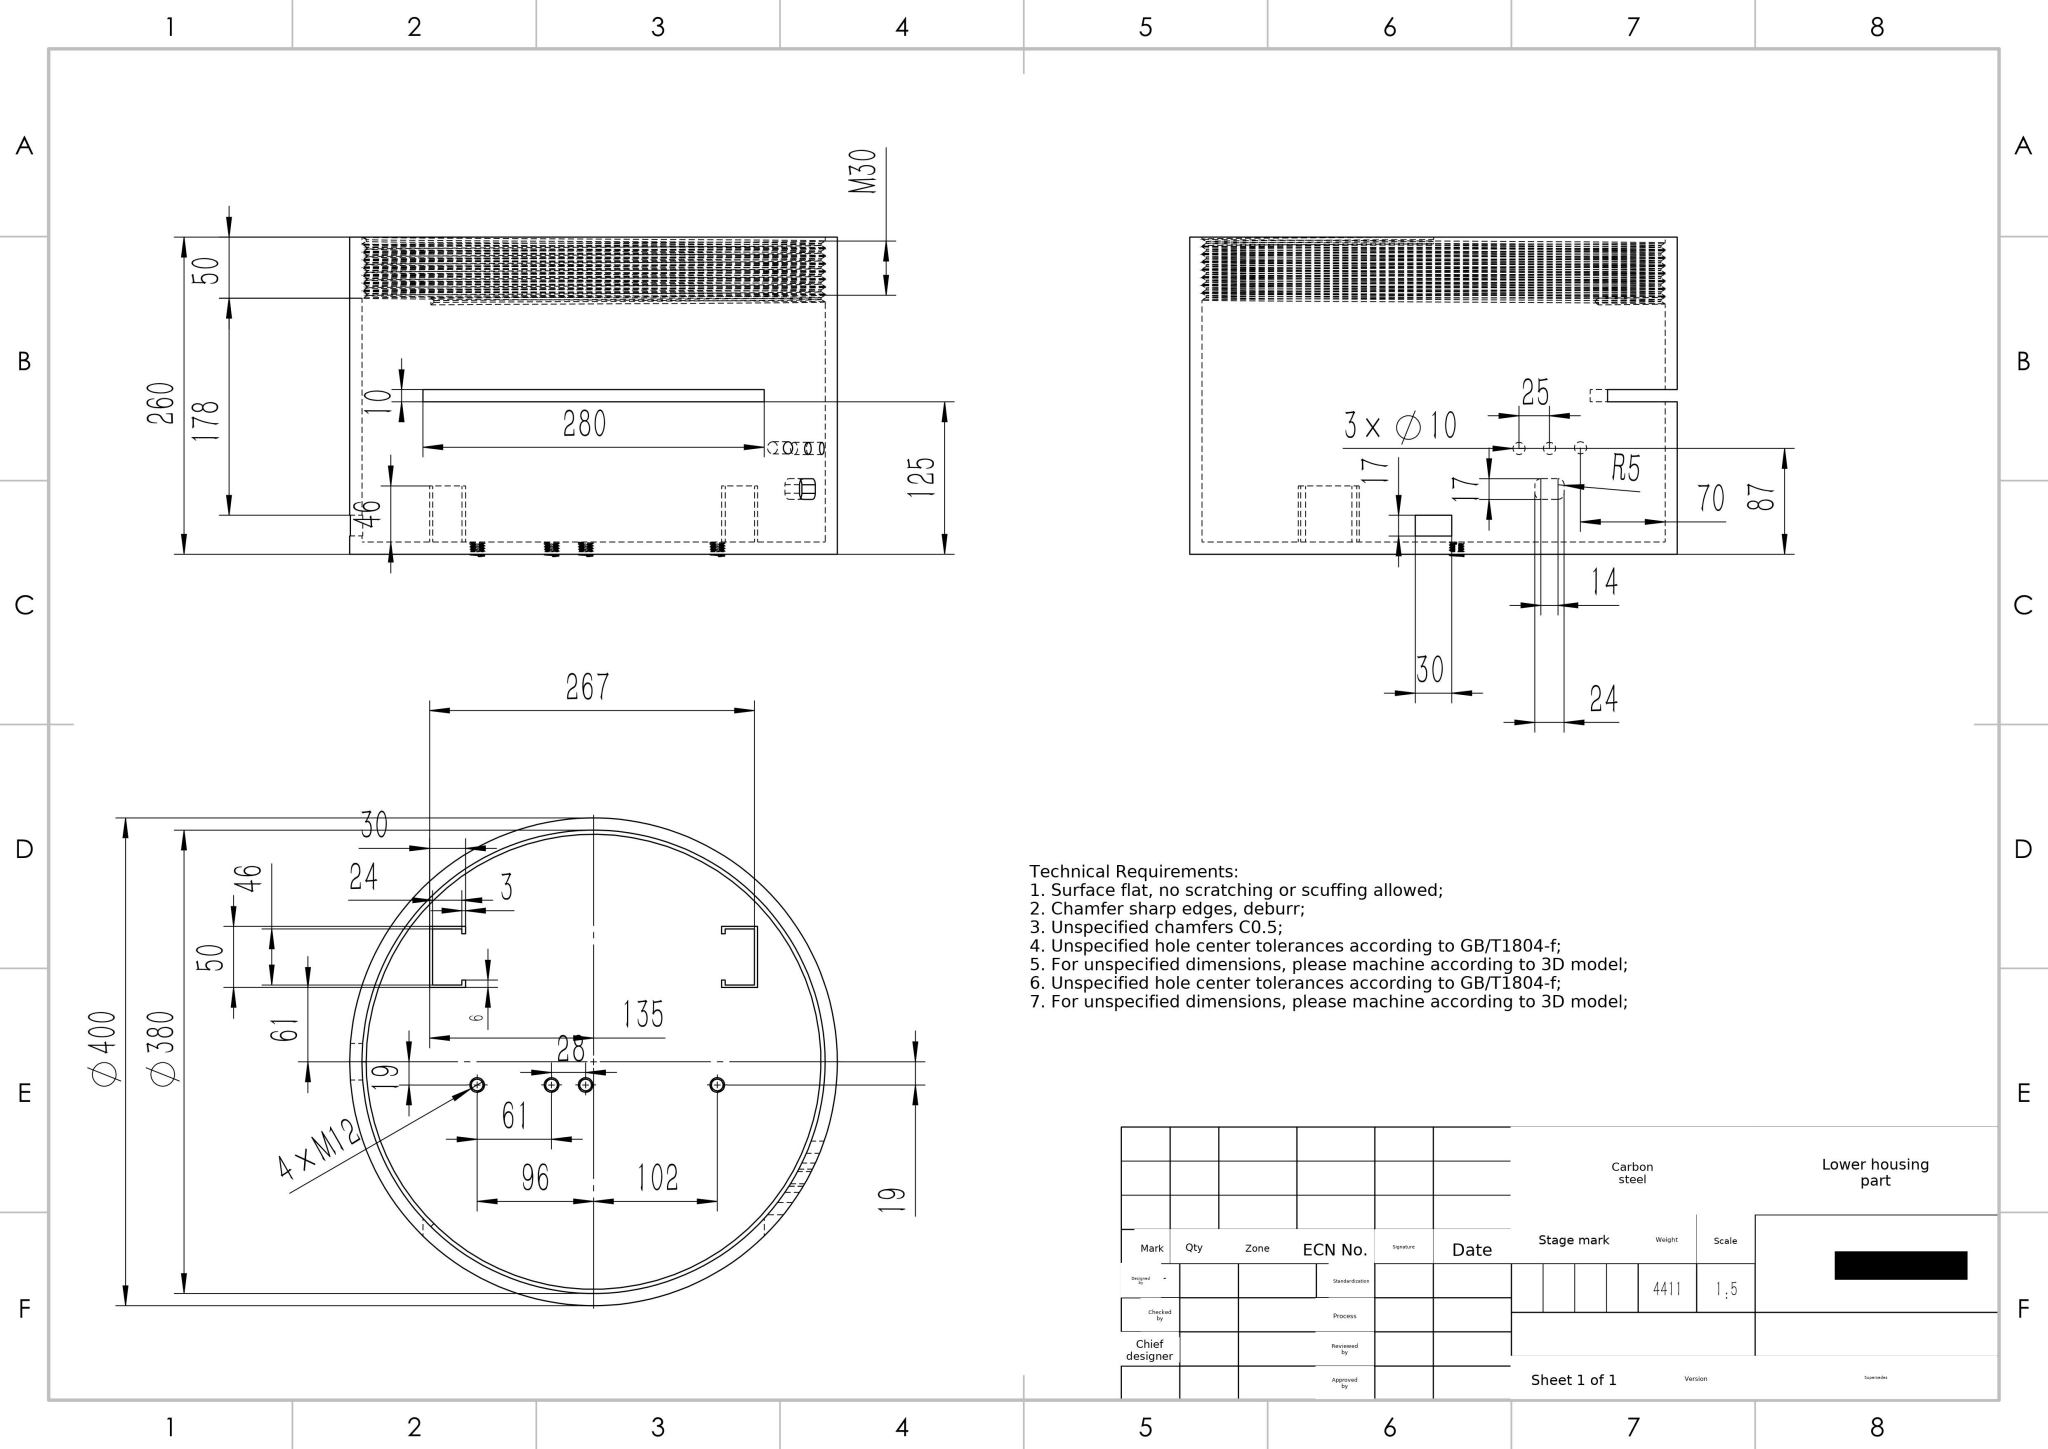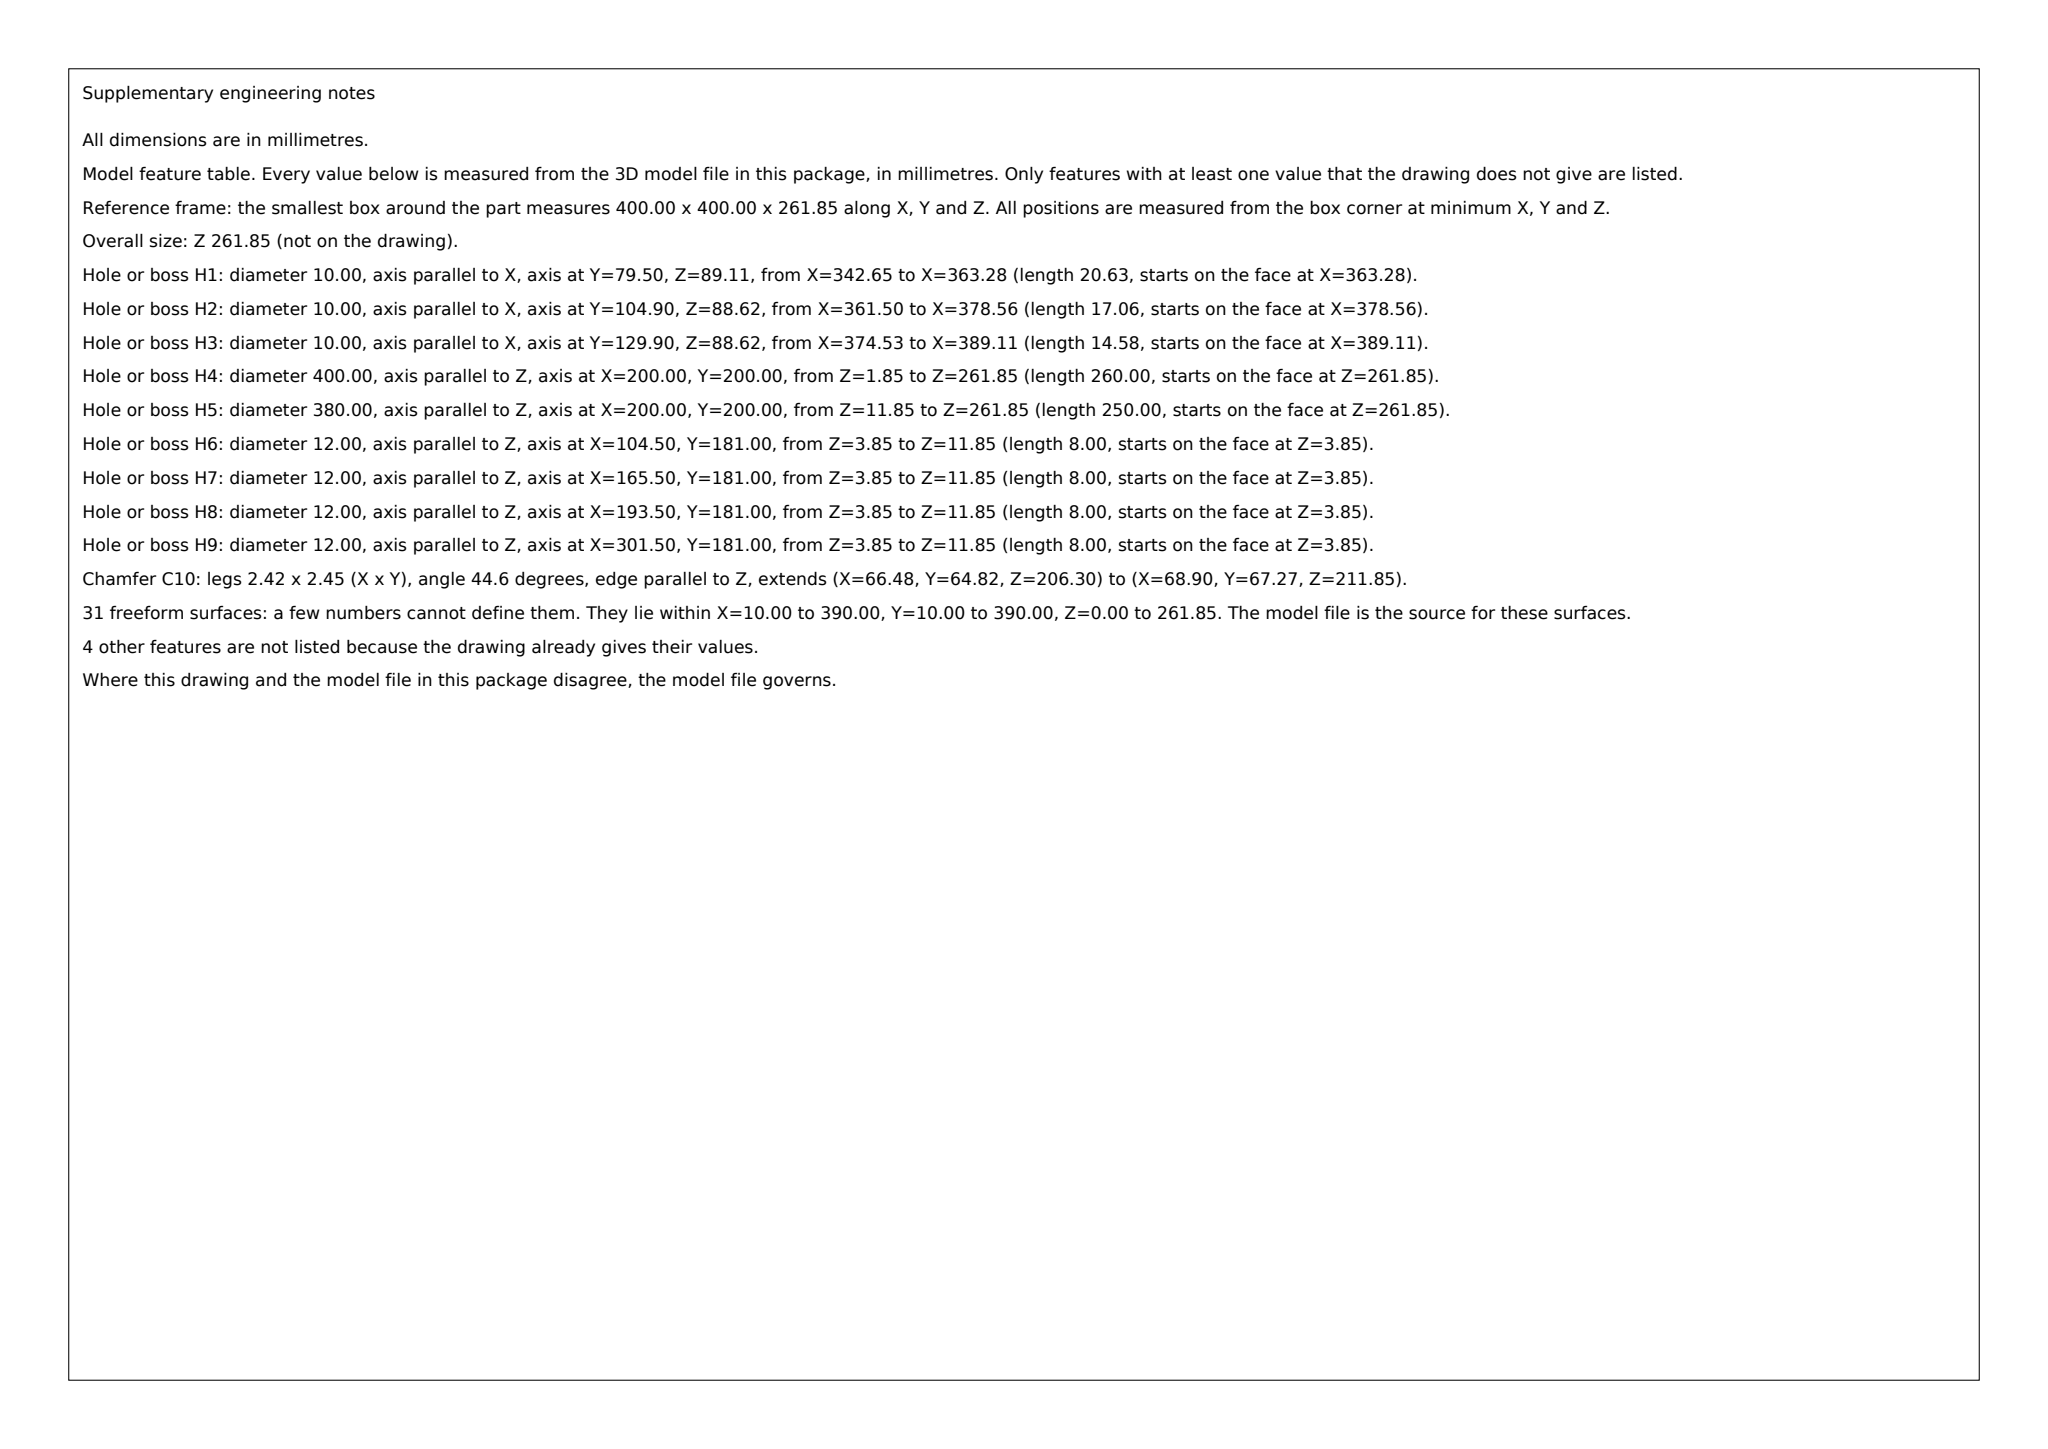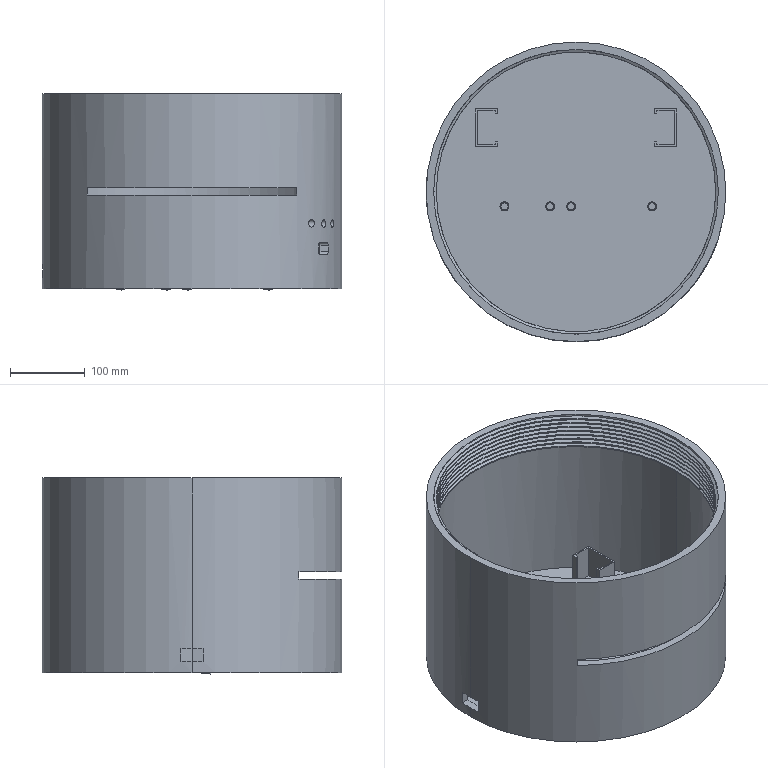Part | SolidWorks | mm | material Carbon steel | 1 solid | 147 faces | box 400 x 400 x 261.85 mm | volume 4412911 mm3 | cylinder 61 | plane 55 | spline 31 | commonest cylinder face diameters 12 x32 380 x17 10 x10 400 x2